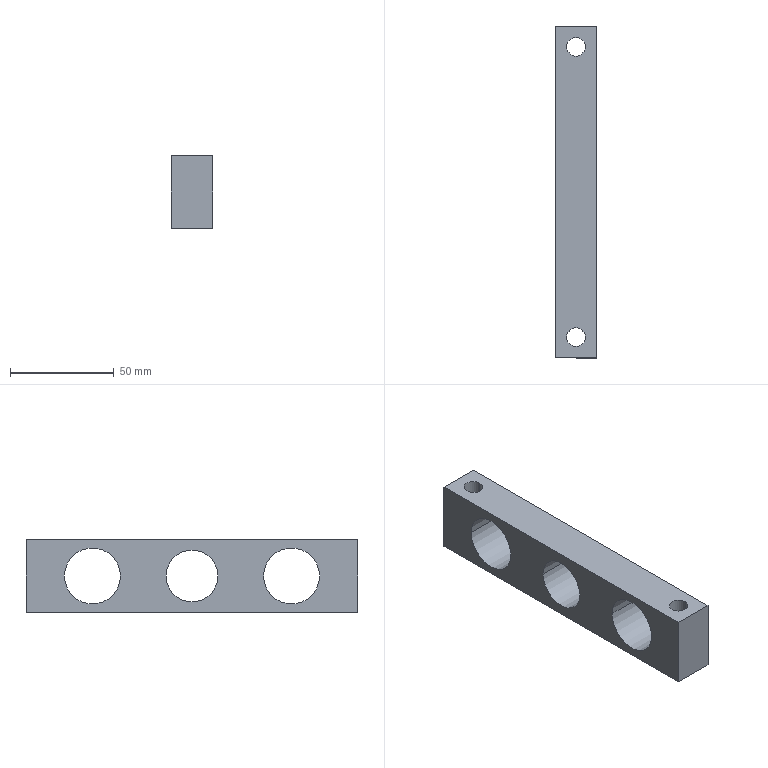Component | SolidWorks | ClampingAssembly-2_CylinderLockingBlock-1 | 1 solid | 22 faces | box 20 x 160 x 35 mm | volume 72882 mm3 | cylinder 14 | plane 8 | commonest cylinder face diameters 15 x4 9 x4 27 x4 25 x2 | material Q235
build123d program:
from build123d import *

# Parameters (mm, degrees)
SKETCH1_W                                       = 160
SKETCH1_H                                       = 35
BOSS_EXTRUDE1_DEPTH                             = 20
SKETCH2_R                                       = 12.5
CUT_EXTRUDE1_DEPTH                              = 85.299
SKETCH3_R                                       = 13.5
CUT_EXTRUDE2_DEPTH                              = 85.299
M8_HEX_SOCKET_HEAD_CAP_SCREW_CBORE1_D           = 9
M8_HEX_SOCKET_HEAD_CAP_SCREW_CBORE1_CBORE_D     = 15
M8_HEX_SOCKET_HEAD_CAP_SCREW_CBORE1_CBORE_DEPTH = 8.6


with BuildPart() as part:
    # Sketch1 → Boss-Extrude1 (new body)
    with BuildSketch(Plane.XY):
        Rectangle(SKETCH1_W, SKETCH1_H)
    extrude(amount=BOSS_EXTRUDE1_DEPTH)

    # Sketch2 → Cut-Extrude1 (cut, through all)
    with BuildSketch(Plane.XY.offset(20)):
        Circle(SKETCH2_R)
    extrude(amount=-CUT_EXTRUDE1_DEPTH, mode=Mode.SUBTRACT)

    # Sketch3 → Cut-Extrude2 (cut, through all)
    with BuildSketch(Plane(origin=(0, 0, 0), x_dir=(-1, 0, 0), z_dir=(0, 0, -1))):
        with Locations((48, 0)):
            Circle(SKETCH3_R)
    cut_extrude2 = extrude(amount=-CUT_EXTRUDE2_DEPTH, mode=Mode.SUBTRACT)

    # Mirror1: Cut-Extrude2 across plane
    add(cut_extrude2.mirror(Plane(origin=(0, 0, 0), x_dir=(0, 0, 1), z_dir=(1, 0, 0))), mode=Mode.SUBTRACT)

    # M8 Hex Socket Head Cap Screw CBORE1 (through all)
    with Locations(Plane(origin=(-70, 17.5, 10), x_dir=(0, 0, 1), z_dir=(0, 1, 0))):
        with Locations((0, 0), (0, 140)):
            CounterBoreHole(M8_HEX_SOCKET_HEAD_CAP_SCREW_CBORE1_D / 2, M8_HEX_SOCKET_HEAD_CAP_SCREW_CBORE1_CBORE_D / 2, M8_HEX_SOCKET_HEAD_CAP_SCREW_CBORE1_CBORE_DEPTH)


solid = part.part

# Placed as in the assembly
solid = solid.moved(Location((-173.215, -26.917, -1210.457), (-90, 90, 0)))
STEP:
#1=COLOUR_RGB('',0.7922,0.8196,0.9333);
#2=FILL_AREA_STYLE_COLOUR('',#1);
#3=FILL_AREA_STYLE('',(#2));
#4=SURFACE_STYLE_FILL_AREA(#3);
#5=SURFACE_SIDE_STYLE('',(#4));
#6=SURFACE_STYLE_USAGE(.BOTH.,#5);
#7=PRESENTATION_STYLE_ASSIGNMENT((#6));
#8=CARTESIAN_POINT('',(-6.721,1.696,-48.006));
#9=VERTEX_POINT('',#8);
#10=CARTESIAN_POINT('',(-6.131,1.696,-48.006));
#11=VERTEX_POINT('',#10);
#12=CARTESIAN_POINT('',(-6.426,1.696,-48.006));
#13=DIRECTION('',(0.,0.,-1.));
#14=DIRECTION('',(1.,-0.,0.));
#15=AXIS2_PLACEMENT_3D('',#12,#13,#14);
#16=CIRCLE('',#15,0.2953);
#17=EDGE_CURVE('',#9,#11,#16,.T.);
#18=ORIENTED_EDGE('',*,*,#17,.F.);
#19=CARTESIAN_POINT('',(-6.721,1.696,-48.345));
#20=VERTEX_POINT('',#19);
#21=CARTESIAN_POINT('',(-6.721,1.696,-48.345));
#22=DIRECTION('',(0.,0.,-1.));
#23=VECTOR('',#22,39.37);
#24=LINE('',#21,#23);
#25=EDGE_CURVE('',#9,#20,#24,.T.);
#26=ORIENTED_EDGE('',*,*,#25,.T.);
#27=CARTESIAN_POINT('',(-6.131,1.696,-48.345));
#28=VERTEX_POINT('',#27);
#29=CARTESIAN_POINT('',(-6.426,1.696,-48.345));
#30=DIRECTION('',(0.,0.,-1.));
#31=DIRECTION('',(1.,-0.,0.));
#32=AXIS2_PLACEMENT_3D('',#29,#30,#31);
#33=CIRCLE('',#32,0.2953);
#34=EDGE_CURVE('',#20,#28,#33,.T.);
#35=ORIENTED_EDGE('',*,*,#34,.T.);
#36=CARTESIAN_POINT('',(-6.131,1.696,-48.345));
#37=DIRECTION('',(0.,0.,-1.));
#38=VECTOR('',#37,39.37);
#39=LINE('',#36,#38);
#40=EDGE_CURVE('',#11,#28,#39,.T.);
#41=ORIENTED_EDGE('',*,*,#40,.F.);
#42=EDGE_LOOP('',(#18,#26,#35,#41));
#43=FACE_OUTER_BOUND('',#42,.T.);
#44=CARTESIAN_POINT('',(-6.426,1.696,-48.345));
#45=DIRECTION('',(0.,0.,-1.));
#46=DIRECTION('',(1.,-0.,0.));
#47=AXIS2_PLACEMENT_3D('',#44,#45,#46);
#48=CYLINDRICAL_SURFACE('',#47,0.2953);
#49=ADVANCED_FACE('',(#43),#48,.F.);
#50=CARTESIAN_POINT('',(-6.603,1.696,-46.967));
#51=VERTEX_POINT('',#50);
#52=CARTESIAN_POINT('',(-6.249,1.696,-46.967));
#53=VERTEX_POINT('',#52);
#54=CARTESIAN_POINT('',(-6.426,1.696,-46.967));
#55=DIRECTION('',(0.,0.,-1.));
#56=DIRECTION('',(1.,0.,0.));
#57=AXIS2_PLACEMENT_3D('',#54,#55,#56);
#58=CIRCLE('',#57,0.1772);
#59=EDGE_CURVE('',#51,#53,#58,.T.);
#60=ORIENTED_EDGE('',*,*,#59,.F.);
#61=CARTESIAN_POINT('',(-6.603,1.696,-48.006));
#62=VERTEX_POINT('',#61);
#63=CARTESIAN_POINT('',(-6.603,1.696,-48.345));
#64=DIRECTION('',(0.,0.,-1.));
#65=VECTOR('',#64,39.37);
#66=LINE('',#63,#65);
#67=EDGE_CURVE('',#51,#62,#66,.T.);
#68=ORIENTED_EDGE('',*,*,#67,.T.);
#69=CARTESIAN_POINT('',(-6.249,1.696,-48.006));
#70=VERTEX_POINT('',#69);
#71=CARTESIAN_POINT('',(-6.426,1.696,-48.006));
#72=DIRECTION('',(0.,0.,-1.));
#73=DIRECTION('',(1.,0.,0.));
#74=AXIS2_PLACEMENT_3D('',#71,#72,#73);
#75=CIRCLE('',#74,0.1772);
#76=EDGE_CURVE('',#62,#70,#75,.T.);
#77=ORIENTED_EDGE('',*,*,#76,.T.);
#78=CARTESIAN_POINT('',(-6.249,1.696,-48.345));
#79=DIRECTION('',(0.,0.,-1.));
#80=VECTOR('',#79,39.37);
#81=LINE('',#78,#80);
#82=EDGE_CURVE('',#53,#70,#81,.T.);
#83=ORIENTED_EDGE('',*,*,#82,.F.);
#84=EDGE_LOOP('',(#60,#68,#77,#83));
#85=FACE_OUTER_BOUND('',#84,.T.);
#86=CARTESIAN_POINT('',(-6.426,1.696,-48.345));
#87=DIRECTION('',(0.,0.,-1.));
#88=DIRECTION('',(1.,0.,0.));
#89=AXIS2_PLACEMENT_3D('',#86,#87,#88);
#90=CYLINDRICAL_SURFACE('',#89,0.1772);
#91=ADVANCED_FACE('',(#85),#90,.F.);
#92=CARTESIAN_POINT('',(-6.721,-3.816,-48.006));
#93=VERTEX_POINT('',#92);
#94=CARTESIAN_POINT('',(-6.131,-3.816,-48.006));
#95=VERTEX_POINT('',#94);
#96=CARTESIAN_POINT('',(-6.426,-3.816,-48.006));
#97=DIRECTION('',(0.,0.,-1.));
#98=DIRECTION('',(1.,0.,0.));
#99=AXIS2_PLACEMENT_3D('',#96,#97,#98);
#100=CIRCLE('',#99,0.2953);
#101=EDGE_CURVE('',#93,#95,#100,.T.);
#102=ORIENTED_EDGE('',*,*,#101,.F.);
#103=CARTESIAN_POINT('',(-6.721,-3.816,-48.345));
#104=VERTEX_POINT('',#103);
#105=CARTESIAN_POINT('',(-6.721,-3.816,-48.345));
#106=DIRECTION('',(0.,0.,-1.));
#107=VECTOR('',#106,39.37);
#108=LINE('',#105,#107);
#109=EDGE_CURVE('',#93,#104,#108,.T.);
#110=ORIENTED_EDGE('',*,*,#109,.T.);
#111=CARTESIAN_POINT('',(-6.131,-3.816,-48.345));
#112=VERTEX_POINT('',#111);
#113=CARTESIAN_POINT('',(-6.426,-3.816,-48.345));
#114=DIRECTION('',(0.,0.,-1.));
#115=DIRECTION('',(1.,0.,0.));
#116=AXIS2_PLACEMENT_3D('',#113,#114,#115);
#117=CIRCLE('',#116,0.2953);
#118=EDGE_CURVE('',#104,#112,#117,.T.);
#119=ORIENTED_EDGE('',*,*,#118,.T.);
#120=CARTESIAN_POINT('',(-6.131,-3.816,-48.345));
#121=DIRECTION('',(0.,0.,-1.));
#122=VECTOR('',#121,39.37);
#123=LINE('',#120,#122);
#124=EDGE_CURVE('',#95,#112,#123,.T.);
#125=ORIENTED_EDGE('',*,*,#124,.F.);
#126=EDGE_LOOP('',(#102,#110,#119,#125));
#127=FACE_OUTER_BOUND('',#126,.T.);
#128=CARTESIAN_POINT('',(-6.426,-3.816,-48.345));
#129=DIRECTION('',(0.,0.,-1.));
#130=DIRECTION('',(1.,0.,0.));
#131=AXIS2_PLACEMENT_3D('',#128,#129,#130);
#132=CYLINDRICAL_SURFACE('',#131,0.2953);
#133=ADVANCED_FACE('',(#127),#132,.F.);
#134=CARTESIAN_POINT('',(-6.603,-3.816,-46.967));
#135=VERTEX_POINT('',#134);
#136=CARTESIAN_POINT('',(-6.249,-3.816,-46.967));
#137=VERTEX_POINT('',#136);
#138=CARTESIAN_POINT('',(-6.426,-3.816,-46.967));
#139=DIRECTION('',(0.,0.,-1.));
#140=DIRECTION('',(1.,0.,0.));
#141=AXIS2_PLACEMENT_3D('',#138,#139,#140);
#142=CIRCLE('',#141,0.1772);
#143=EDGE_CURVE('',#135,#137,#142,.T.);
#144=ORIENTED_EDGE('',*,*,#143,.F.);
#145=CARTESIAN_POINT('',(-6.603,-3.816,-48.006));
#146=VERTEX_POINT('',#145);
#147=CARTESIAN_POINT('',(-6.603,-3.816,-48.345));
#148=DIRECTION('',(0.,0.,-1.));
#149=VECTOR('',#148,39.37);
#150=LINE('',#147,#149);
#151=EDGE_CURVE('',#135,#146,#150,.T.);
#152=ORIENTED_EDGE('',*,*,#151,.T.);
#153=CARTESIAN_POINT('',(-6.249,-3.816,-48.006));
#154=VERTEX_POINT('',#153);
#155=CARTESIAN_POINT('',(-6.426,-3.816,-48.006));
#156=DIRECTION('',(0.,0.,-1.));
#157=DIRECTION('',(1.,0.,0.));
#158=AXIS2_PLACEMENT_3D('',#155,#156,#157);
#159=CIRCLE('',#158,0.1772);
#160=EDGE_CURVE('',#146,#154,#159,.T.);
#161=ORIENTED_EDGE('',*,*,#160,.T.);
#162=CARTESIAN_POINT('',(-6.249,-3.816,-48.345));
#163=DIRECTION('',(0.,0.,-1.));
#164=VECTOR('',#163,39.37);
#165=LINE('',#162,#164);
#166=EDGE_CURVE('',#137,#154,#165,.T.);
#167=ORIENTED_EDGE('',*,*,#166,.F.);
#168=EDGE_LOOP('',(#144,#152,#161,#167));
#169=FACE_OUTER_BOUND('',#168,.T.);
#170=CARTESIAN_POINT('',(-6.426,-3.816,-48.345));
#171=DIRECTION('',(0.,0.,-1.));
#172=DIRECTION('',(1.,0.,0.));
#173=AXIS2_PLACEMENT_3D('',#170,#171,#172);
#174=CYLINDRICAL_SURFACE('',#173,0.1772);
#175=ADVANCED_FACE('',(#169),#174,.F.);
#176=CARTESIAN_POINT('',(-6.032,-2.418,-47.656));
#177=VERTEX_POINT('',#176);
#178=CARTESIAN_POINT('',(-6.032,-3.481,-47.656));
#179=VERTEX_POINT('',#178);
#180=CARTESIAN_POINT('',(-6.032,-2.949,-47.656));
#181=DIRECTION('',(1.,-0.,0.));
#182=DIRECTION('',(0.,-1.,0.));
#183=AXIS2_PLACEMENT_3D('',#180,#181,#182);
#184=CIRCLE('',#183,0.5315);
#185=EDGE_CURVE('',#177,#179,#184,.T.);
#186=ORIENTED_EDGE('',*,*,#185,.T.);
#187=CARTESIAN_POINT('',(-6.819,-3.481,-47.656));
#188=VERTEX_POINT('',#187);
#189=CARTESIAN_POINT('',(-6.032,-3.481,-47.656));
#190=DIRECTION('',(-1.,0.,-0.));
#191=VECTOR('',#190,39.37);
#192=LINE('',#189,#191);
#193=EDGE_CURVE('',#179,#188,#192,.T.);
#194=ORIENTED_EDGE('',*,*,#193,.T.);
#195=CARTESIAN_POINT('',(-6.819,-2.418,-47.656));
#196=VERTEX_POINT('',#195);
#197=CARTESIAN_POINT('',(-6.819,-2.949,-47.656));
#198=DIRECTION('',(1.,-0.,0.));
#199=DIRECTION('',(0.,-1.,0.));
#200=AXIS2_PLACEMENT_3D('',#197,#198,#199);
#201=CIRCLE('',#200,0.5315);
#202=EDGE_CURVE('',#196,#188,#201,.T.);
#203=ORIENTED_EDGE('',*,*,#202,.F.);
#204=CARTESIAN_POINT('',(-6.032,-2.418,-47.656));
#205=DIRECTION('',(-1.,0.,-0.));
#206=VECTOR('',#205,39.37);
#207=LINE('',#204,#206);
#208=EDGE_CURVE('',#177,#196,#207,.T.);
#209=ORIENTED_EDGE('',*,*,#208,.F.);
#210=EDGE_LOOP('',(#186,#194,#203,#209));
#211=FACE_OUTER_BOUND('',#210,.T.);
#212=CARTESIAN_POINT('',(-6.032,-2.949,-47.656));
#213=DIRECTION('',(-1.,0.,-0.));
#214=DIRECTION('',(0.,1.,0.));
#215=AXIS2_PLACEMENT_3D('',#212,#213,#214);
#216=CYLINDRICAL_SURFACE('',#215,0.5315);
#217=ADVANCED_FACE('',(#211),#216,.F.);
#218=CARTESIAN_POINT('',(-6.032,0.2985,-47.656));
#219=VERTEX_POINT('',#218);
#220=CARTESIAN_POINT('',(-6.032,1.362,-47.656));
#221=VERTEX_POINT('',#220);
#222=CARTESIAN_POINT('',(-6.032,0.83,-47.656));
#223=DIRECTION('',(-1.,0.,-0.));
#224=DIRECTION('',(0.,1.,0.));
#225=AXIS2_PLACEMENT_3D('',#222,#223,#224);
#226=CIRCLE('',#225,0.5315);
#227=EDGE_CURVE('',#219,#221,#226,.T.);
#228=ORIENTED_EDGE('',*,*,#227,.F.);
#229=CARTESIAN_POINT('',(-6.819,0.2985,-47.656));
#230=VERTEX_POINT('',#229);
#231=CARTESIAN_POINT('',(-6.032,0.2985,-47.656));
#232=DIRECTION('',(-1.,0.,-0.));
#233=VECTOR('',#232,39.37);
#234=LINE('',#231,#233);
#235=EDGE_CURVE('',#219,#230,#234,.T.);
#236=ORIENTED_EDGE('',*,*,#235,.T.);
#237=CARTESIAN_POINT('',(-6.819,1.362,-47.656));
#238=VERTEX_POINT('',#237);
#239=CARTESIAN_POINT('',(-6.819,0.83,-47.656));
#240=DIRECTION('',(-1.,0.,-0.));
#241=DIRECTION('',(0.,1.,0.));
#242=AXIS2_PLACEMENT_3D('',#239,#240,#241);
#243=CIRCLE('',#242,0.5315);
#244=EDGE_CURVE('',#230,#238,#243,.T.);
#245=ORIENTED_EDGE('',*,*,#244,.T.);
#246=CARTESIAN_POINT('',(-6.032,1.362,-47.656));
#247=DIRECTION('',(-1.,0.,-0.));
#248=VECTOR('',#247,39.37);
#249=LINE('',#246,#248);
#250=EDGE_CURVE('',#221,#238,#249,.T.);
#251=ORIENTED_EDGE('',*,*,#250,.F.);
#252=EDGE_LOOP('',(#228,#236,#245,#251));
#253=FACE_OUTER_BOUND('',#252,.T.);
#254=CARTESIAN_POINT('',(-6.032,0.83,-47.656));
#255=DIRECTION('',(-1.,0.,-0.));
#256=DIRECTION('',(0.,1.,0.));
#257=AXIS2_PLACEMENT_3D('',#254,#255,#256);
#258=CYLINDRICAL_SURFACE('',#257,0.5315);
#259=ADVANCED_FACE('',(#253),#258,.F.);
#260=CARTESIAN_POINT('',(-6.819,-0.5676,-47.656));
#261=VERTEX_POINT('',#260);
#262=CARTESIAN_POINT('',(-6.819,-1.552,-47.656));
#263=VERTEX_POINT('',#262);
#264=CARTESIAN_POINT('',(-6.819,-1.06,-47.656));
#265=DIRECTION('',(1.,-0.,0.));
#266=DIRECTION('',(0.,-1.,0.));
#267=AXIS2_PLACEMENT_3D('',#264,#265,#266);
#268=CIRCLE('',#267,0.4921);
#269=EDGE_CURVE('',#261,#263,#268,.T.);
#270=ORIENTED_EDGE('',*,*,#269,.F.);
#271=CARTESIAN_POINT('',(-6.032,-0.5676,-47.656));
#272=VERTEX_POINT('',#271);
#273=CARTESIAN_POINT('',(-6.819,-0.5676,-47.656));
#274=DIRECTION('',(1.,-0.,0.));
#275=VECTOR('',#274,39.37);
#276=LINE('',#273,#275);
#277=EDGE_CURVE('',#261,#272,#276,.T.);
#278=ORIENTED_EDGE('',*,*,#277,.T.);
#279=CARTESIAN_POINT('',(-6.032,-1.552,-47.656));
#280=VERTEX_POINT('',#279);
#281=CARTESIAN_POINT('',(-6.032,-1.06,-47.656));
#282=DIRECTION('',(1.,-0.,0.));
#283=DIRECTION('',(0.,-1.,0.));
#284=AXIS2_PLACEMENT_3D('',#281,#282,#283);
#285=CIRCLE('',#284,0.4921);
#286=EDGE_CURVE('',#272,#280,#285,.T.);
#287=ORIENTED_EDGE('',*,*,#286,.T.);
#288=CARTESIAN_POINT('',(-6.819,-1.552,-47.656));
#289=DIRECTION('',(1.,-0.,0.));
#290=VECTOR('',#289,39.37);
#291=LINE('',#288,#290);
#292=EDGE_CURVE('',#263,#280,#291,.T.);
#293=ORIENTED_EDGE('',*,*,#292,.F.);
#294=EDGE_LOOP('',(#270,#278,#287,#293));
#295=FACE_OUTER_BOUND('',#294,.T.);
#296=CARTESIAN_POINT('',(-6.819,-1.06,-47.656));
#297=DIRECTION('',(1.,-0.,0.));
#298=DIRECTION('',(0.,-1.,0.));
#299=AXIS2_PLACEMENT_3D('',#296,#297,#298);
#300=CYLINDRICAL_SURFACE('',#299,0.4921);
#301=ADVANCED_FACE('',(#295),#300,.F.);
#302=CARTESIAN_POINT('',(-6.032,-4.209,-46.967));
#303=VERTEX_POINT('',#302);
#304=CARTESIAN_POINT('',(-6.032,-4.209,-48.345));
#305=VERTEX_POINT('',#304);
#306=CARTESIAN_POINT('',(-6.032,-4.209,-48.345));
#307=DIRECTION('',(0.,0.,-1.));
#308=VECTOR('',#307,39.37);
#309=LINE('',#306,#308);
#310=EDGE_CURVE('',#303,#305,#309,.T.);
#311=ORIENTED_EDGE('',*,*,#310,.T.);
#312=CARTESIAN_POINT('',(-6.032,2.09,-48.345));
#313=VERTEX_POINT('',#312);
#314=CARTESIAN_POINT('',(-6.032,2.09,-48.345));
#315=DIRECTION('',(0.,1.,0.));
#316=VECTOR('',#315,39.37);
#317=LINE('',#314,#316);
#318=EDGE_CURVE('',#305,#313,#317,.T.);
#319=ORIENTED_EDGE('',*,*,#318,.T.);
#320=CARTESIAN_POINT('',(-6.032,2.09,-46.967));
#321=VERTEX_POINT('',#320);
#322=CARTESIAN_POINT('',(-6.032,2.09,-48.345));
#323=DIRECTION('',(-0.,-0.,1.));
#324=VECTOR('',#323,39.37);
#325=LINE('',#322,#324);
#326=EDGE_CURVE('',#313,#321,#325,.T.);
#327=ORIENTED_EDGE('',*,*,#326,.T.);
#328=CARTESIAN_POINT('',(-6.032,2.09,-46.967));
#329=DIRECTION('',(-0.,-1.,-0.));
#330=VECTOR('',#329,39.37);
#331=LINE('',#328,#330);
#332=EDGE_CURVE('',#321,#303,#331,.T.);
#333=ORIENTED_EDGE('',*,*,#332,.T.);
#334=EDGE_LOOP('',(#311,#319,#327,#333));
#335=FACE_OUTER_BOUND('',#334,.T.);
#336=CARTESIAN_POINT('',(-6.032,-1.06,-47.656));
#337=DIRECTION('',(1.,-0.,0.));
#338=DIRECTION('',(0.,-1.,0.));
#339=AXIS2_PLACEMENT_3D('',#336,#337,#338);
#340=CIRCLE('',#339,0.4921);
#341=EDGE_CURVE('',#280,#272,#340,.T.);
#342=ORIENTED_EDGE('',*,*,#341,.F.);
#343=ORIENTED_EDGE('',*,*,#286,.F.);
#344=EDGE_LOOP('',(#342,#343));
#345=FACE_BOUND('',#344,.T.);
#346=CARTESIAN_POINT('',(-6.032,0.83,-47.656));
#347=DIRECTION('',(-1.,0.,-0.));
#348=DIRECTION('',(0.,1.,0.));
#349=AXIS2_PLACEMENT_3D('',#346,#347,#348);
#350=CIRCLE('',#349,0.5315);
#351=EDGE_CURVE('',#221,#219,#350,.T.);
#352=ORIENTED_EDGE('',*,*,#351,.T.);
#353=ORIENTED_EDGE('',*,*,#227,.T.);
#354=EDGE_LOOP('',(#352,#353));
#355=FACE_BOUND('',#354,.T.);
#356=ORIENTED_EDGE('',*,*,#185,.F.);
#357=CARTESIAN_POINT('',(-6.032,-2.949,-47.656));
#358=DIRECTION('',(1.,-0.,0.));
#359=DIRECTION('',(0.,-1.,0.));
#360=AXIS2_PLACEMENT_3D('',#357,#358,#359);
#361=CIRCLE('',#360,0.5315);
#362=EDGE_CURVE('',#179,#177,#361,.T.);
#363=ORIENTED_EDGE('',*,*,#362,.F.);
#364=EDGE_LOOP('',(#356,#363));
#365=FACE_BOUND('',#364,.T.);
#366=CARTESIAN_POINT('',(-6.032,-1.06,-47.656));
#367=DIRECTION('',(1.,-0.,0.));
#368=DIRECTION('',(-0.,-1.,-0.));
#369=AXIS2_PLACEMENT_3D('',#366,#367,#368);
#370=PLANE('',#369);
#371=ADVANCED_FACE('',(#335,#345,#355,#365),#370,.T.);
#372=CARTESIAN_POINT('',(-6.819,-4.209,-46.967));
#373=VERTEX_POINT('',#372);
#374=CARTESIAN_POINT('',(-6.819,-4.209,-48.345));
#375=VERTEX_POINT('',#374);
#376=CARTESIAN_POINT('',(-6.819,-4.209,-48.345));
#377=DIRECTION('',(0.,0.,-1.));
#378=VECTOR('',#377,39.37);
#379=LINE('',#376,#378);
#380=EDGE_CURVE('',#373,#375,#379,.T.);
#381=ORIENTED_EDGE('',*,*,#380,.F.);
#382=CARTESIAN_POINT('',(-6.819,2.09,-46.967));
#383=VERTEX_POINT('',#382);
#384=CARTESIAN_POINT('',(-6.819,2.09,-46.967));
#385=DIRECTION('',(-0.,-1.,-0.));
#386=VECTOR('',#385,39.37);
#387=LINE('',#384,#386);
#388=EDGE_CURVE('',#383,#373,#387,.T.);
#389=ORIENTED_EDGE('',*,*,#388,.F.);
#390=CARTESIAN_POINT('',(-6.819,2.09,-48.345));
#391=VERTEX_POINT('',#390);
#392=CARTESIAN_POINT('',(-6.819,2.09,-48.345));
#393=DIRECTION('',(-0.,-0.,1.));
#394=VECTOR('',#393,39.37);
#395=LINE('',#392,#394);
#396=EDGE_CURVE('',#391,#383,#395,.T.);
#397=ORIENTED_EDGE('',*,*,#396,.F.);
#398=CARTESIAN_POINT('',(-6.819,2.09,-48.345));
#399=DIRECTION('',(0.,1.,0.));
#400=VECTOR('',#399,39.37);
#401=LINE('',#398,#400);
#402=EDGE_CURVE('',#375,#391,#401,.T.);
#403=ORIENTED_EDGE('',*,*,#402,.F.);
#404=EDGE_LOOP('',(#381,#389,#397,#403));
#405=FACE_OUTER_BOUND('',#404,.T.);
#406=CARTESIAN_POINT('',(-6.819,-1.06,-47.656));
#407=DIRECTION('',(1.,-0.,0.));
#408=DIRECTION('',(0.,-1.,0.));
#409=AXIS2_PLACEMENT_3D('',#406,#407,#408);
#410=CIRCLE('',#409,0.4921);
#411=EDGE_CURVE('',#263,#261,#410,.T.);
#412=ORIENTED_EDGE('',*,*,#411,.T.);
#413=ORIENTED_EDGE('',*,*,#269,.T.);
#414=EDGE_LOOP('',(#412,#413));
#415=FACE_BOUND('',#414,.T.);
#416=CARTESIAN_POINT('',(-6.819,0.83,-47.656));
#417=DIRECTION('',(-1.,0.,-0.));
#418=DIRECTION('',(0.,1.,0.));
#419=AXIS2_PLACEMENT_3D('',#416,#417,#418);
#420=CIRCLE('',#419,0.5315);
#421=EDGE_CURVE('',#238,#230,#420,.T.);
#422=ORIENTED_EDGE('',*,*,#421,.F.);
#423=ORIENTED_EDGE('',*,*,#244,.F.);
#424=EDGE_LOOP('',(#422,#423));
#425=FACE_BOUND('',#424,.T.);
#426=ORIENTED_EDGE('',*,*,#202,.T.);
#427=CARTESIAN_POINT('',(-6.819,-2.949,-47.656));
#428=DIRECTION('',(1.,-0.,0.));
#429=DIRECTION('',(0.,-1.,0.));
#430=AXIS2_PLACEMENT_3D('',#427,#428,#429);
#431=CIRCLE('',#430,0.5315);
#432=EDGE_CURVE('',#188,#196,#431,.T.);
#433=ORIENTED_EDGE('',*,*,#432,.T.);
#434=EDGE_LOOP('',(#426,#433));
#435=FACE_BOUND('',#434,.T.);
#436=CARTESIAN_POINT('',(-6.819,-1.06,-47.656));
#437=DIRECTION('',(1.,-0.,0.));
#438=DIRECTION('',(-0.,-1.,-0.));
#439=AXIS2_PLACEMENT_3D('',#436,#437,#438);
#440=PLANE('',#439);
#441=ADVANCED_FACE('',(#405,#415,#425,#435),#440,.F.);
#442=ORIENTED_EDGE('',*,*,#380,.T.);
#443=CARTESIAN_POINT('',(-6.032,-4.209,-48.345));
#444=DIRECTION('',(-1.,0.,-0.));
#445=VECTOR('',#444,39.37);
#446=LINE('',#443,#445);
#447=EDGE_CURVE('',#305,#375,#446,.T.);
#448=ORIENTED_EDGE('',*,*,#447,.F.);
#449=ORIENTED_EDGE('',*,*,#310,.F.);
#450=CARTESIAN_POINT('',(-6.032,-4.209,-46.967));
#451=DIRECTION('',(-1.,0.,-0.));
#452=VECTOR('',#451,39.37);
#453=LINE('',#450,#452);
#454=EDGE_CURVE('',#303,#373,#453,.T.);
#455=ORIENTED_EDGE('',*,*,#454,.T.);
#456=EDGE_LOOP('',(#442,#448,#449,#455));
#457=FACE_OUTER_BOUND('',#456,.T.);
#458=CARTESIAN_POINT('',(-6.032,-4.209,-48.345));
#459=DIRECTION('',(0.,1.,0.));
#460=DIRECTION('',(1.,-0.,0.));
#461=AXIS2_PLACEMENT_3D('',#458,#459,#460);
#462=PLANE('',#461);
#463=ADVANCED_FACE('',(#457),#462,.F.);
#464=CARTESIAN_POINT('',(-6.426,1.696,-48.345));
#465=DIRECTION('',(0.,0.,-1.));
#466=DIRECTION('',(1.,-0.,0.));
#467=AXIS2_PLACEMENT_3D('',#464,#465,#466);
#468=CIRCLE('',#467,0.2953);
#469=EDGE_CURVE('',#28,#20,#468,.T.);
#470=ORIENTED_EDGE('',*,*,#469,.F.);
#471=ORIENTED_EDGE('',*,*,#34,.F.);
#472=EDGE_LOOP('',(#470,#471));
#473=FACE_BOUND('',#472,.T.);
#474=CARTESIAN_POINT('',(-6.426,-3.816,-48.345));
#475=DIRECTION('',(0.,0.,-1.));
#476=DIRECTION('',(1.,0.,0.));
#477=AXIS2_PLACEMENT_3D('',#474,#475,#476);
#478=CIRCLE('',#477,0.2953);
#479=EDGE_CURVE('',#112,#104,#478,.T.);
#480=ORIENTED_EDGE('',*,*,#479,.F.);
#481=ORIENTED_EDGE('',*,*,#118,.F.);
#482=EDGE_LOOP('',(#480,#481));
#483=FACE_BOUND('',#482,.T.);
#484=ORIENTED_EDGE('',*,*,#402,.T.);
#485=CARTESIAN_POINT('',(-6.032,2.09,-48.345));
#486=DIRECTION('',(-1.,0.,-0.));
#487=VECTOR('',#486,39.37);
#488=LINE('',#485,#487);
#489=EDGE_CURVE('',#313,#391,#488,.T.);
#490=ORIENTED_EDGE('',*,*,#489,.F.);
#491=ORIENTED_EDGE('',*,*,#318,.F.);
#492=ORIENTED_EDGE('',*,*,#447,.T.);
#493=EDGE_LOOP('',(#484,#490,#491,#492));
#494=FACE_OUTER_BOUND('',#493,.T.);
#495=CARTESIAN_POINT('',(-6.032,2.09,-48.345));
#496=DIRECTION('',(-0.,-0.,1.));
#497=DIRECTION('',(-1.,0.,-0.));
#498=AXIS2_PLACEMENT_3D('',#495,#496,#497);
#499=PLANE('',#498);
#500=ADVANCED_FACE('',(#473,#483,#494),#499,.F.);
#501=ORIENTED_EDGE('',*,*,#396,.T.);
#502=CARTESIAN_POINT('',(-6.032,2.09,-46.967));
#503=DIRECTION('',(-1.,0.,-0.));
#504=VECTOR('',#503,39.37);
#505=LINE('',#502,#504);
#506=EDGE_CURVE('',#321,#383,#505,.T.);
#507=ORIENTED_EDGE('',*,*,#506,.F.);
#508=ORIENTED_EDGE('',*,*,#326,.F.);
#509=ORIENTED_EDGE('',*,*,#489,.T.);
#510=EDGE_LOOP('',(#501,#507,#508,#509));
#511=FACE_OUTER_BOUND('',#510,.T.);
#512=CARTESIAN_POINT('',(-6.032,2.09,-48.345));
#513=DIRECTION('',(-0.,-1.,-0.));
#514=DIRECTION('',(-1.,0.,-0.));
#515=AXIS2_PLACEMENT_3D('',#512,#513,#514);
#516=PLANE('',#515);
#517=ADVANCED_FACE('',(#511),#516,.F.);
#518=CARTESIAN_POINT('',(-6.426,1.696,-46.967));
#519=DIRECTION('',(0.,0.,-1.));
#520=DIRECTION('',(1.,0.,0.));
#521=AXIS2_PLACEMENT_3D('',#518,#519,#520);
#522=CIRCLE('',#521,0.1772);
#523=EDGE_CURVE('',#53,#51,#522,.T.);
#524=ORIENTED_EDGE('',*,*,#523,.T.);
#525=ORIENTED_EDGE('',*,*,#59,.T.);
#526=EDGE_LOOP('',(#524,#525));
#527=FACE_BOUND('',#526,.T.);
#528=CARTESIAN_POINT('',(-6.426,-3.816,-46.967));
#529=DIRECTION('',(0.,0.,-1.));
#530=DIRECTION('',(1.,0.,0.));
#531=AXIS2_PLACEMENT_3D('',#528,#529,#530);
#532=CIRCLE('',#531,0.1772);
#533=EDGE_CURVE('',#137,#135,#532,.T.);
#534=ORIENTED_EDGE('',*,*,#533,.T.);
#535=ORIENTED_EDGE('',*,*,#143,.T.);
#536=EDGE_LOOP('',(#534,#535));
#537=FACE_BOUND('',#536,.T.);
#538=ORIENTED_EDGE('',*,*,#388,.T.);
#539=ORIENTED_EDGE('',*,*,#454,.F.);
#540=ORIENTED_EDGE('',*,*,#332,.F.);
#541=ORIENTED_EDGE('',*,*,#506,.T.);
#542=EDGE_LOOP('',(#538,#539,#540,#541));
#543=FACE_OUTER_BOUND('',#542,.T.);
#544=CARTESIAN_POINT('',(-6.032,2.09,-46.967));
#545=DIRECTION('',(0.,0.,-1.));
#546=DIRECTION('',(1.,-0.,0.));
#547=AXIS2_PLACEMENT_3D('',#544,#545,#546);
#548=PLANE('',#547);
#549=ADVANCED_FACE('',(#527,#537,#543),#548,.F.);
#550=ORIENTED_EDGE('',*,*,#277,.F.);
#551=ORIENTED_EDGE('',*,*,#411,.F.);
#552=ORIENTED_EDGE('',*,*,#292,.T.);
#553=ORIENTED_EDGE('',*,*,#341,.T.);
#554=EDGE_LOOP('',(#550,#551,#552,#553));
#555=FACE_OUTER_BOUND('',#554,.T.);
#556=CARTESIAN_POINT('',(-6.819,-1.06,-47.656));
#557=DIRECTION('',(1.,-0.,0.));
#558=DIRECTION('',(0.,-1.,0.));
#559=AXIS2_PLACEMENT_3D('',#556,#557,#558);
#560=CYLINDRICAL_SURFACE('',#559,0.4921);
#561=ADVANCED_FACE('',(#555),#560,.F.);
#562=ORIENTED_EDGE('',*,*,#235,.F.);
#563=ORIENTED_EDGE('',*,*,#351,.F.);
#564=ORIENTED_EDGE('',*,*,#250,.T.);
#565=ORIENTED_EDGE('',*,*,#421,.T.);
#566=EDGE_LOOP('',(#562,#563,#564,#565));
#567=FACE_OUTER_BOUND('',#566,.T.);
#568=CARTESIAN_POINT('',(-6.032,0.83,-47.656));
#569=DIRECTION('',(-1.,0.,-0.));
#570=DIRECTION('',(0.,1.,0.));
#571=AXIS2_PLACEMENT_3D('',#568,#569,#570);
#572=CYLINDRICAL_SURFACE('',#571,0.5315);
#573=ADVANCED_FACE('',(#567),#572,.F.);
#574=ORIENTED_EDGE('',*,*,#193,.F.);
#575=ORIENTED_EDGE('',*,*,#362,.T.);
#576=ORIENTED_EDGE('',*,*,#208,.T.);
#577=ORIENTED_EDGE('',*,*,#432,.F.);
#578=EDGE_LOOP('',(#574,#575,#576,#577));
#579=FACE_OUTER_BOUND('',#578,.T.);
#580=CARTESIAN_POINT('',(-6.032,-2.949,-47.656));
#581=DIRECTION('',(-1.,0.,-0.));
#582=DIRECTION('',(0.,1.,0.));
#583=AXIS2_PLACEMENT_3D('',#580,#581,#582);
#584=CYLINDRICAL_SURFACE('',#583,0.5315);
#585=ADVANCED_FACE('',(#579),#584,.F.);
#586=ORIENTED_EDGE('',*,*,#151,.F.);
#587=ORIENTED_EDGE('',*,*,#533,.F.);
#588=ORIENTED_EDGE('',*,*,#166,.T.);
#589=CARTESIAN_POINT('',(-6.426,-3.816,-48.006));
#590=DIRECTION('',(0.,0.,-1.));
#591=DIRECTION('',(1.,0.,0.));
#592=AXIS2_PLACEMENT_3D('',#589,#590,#591);
#593=CIRCLE('',#592,0.1772);
#594=EDGE_CURVE('',#154,#146,#593,.T.);
#595=ORIENTED_EDGE('',*,*,#594,.T.);
#596=EDGE_LOOP('',(#586,#587,#588,#595));
#597=FACE_OUTER_BOUND('',#596,.T.);
#598=CARTESIAN_POINT('',(-6.426,-3.816,-48.345));
#599=DIRECTION('',(0.,0.,-1.));
#600=DIRECTION('',(1.,0.,0.));
#601=AXIS2_PLACEMENT_3D('',#598,#599,#600);
#602=CYLINDRICAL_SURFACE('',#601,0.1772);
#603=ADVANCED_FACE('',(#597),#602,.F.);
#604=ORIENTED_EDGE('',*,*,#594,.F.);
#605=ORIENTED_EDGE('',*,*,#160,.F.);
#606=EDGE_LOOP('',(#604,#605));
#607=FACE_BOUND('',#606,.T.);
#608=CARTESIAN_POINT('',(-6.426,-3.816,-48.006));
#609=DIRECTION('',(0.,0.,-1.));
#610=DIRECTION('',(1.,0.,0.));
#611=AXIS2_PLACEMENT_3D('',#608,#609,#610);
#612=CIRCLE('',#611,0.2953);
#613=EDGE_CURVE('',#95,#93,#612,.T.);
#614=ORIENTED_EDGE('',*,*,#613,.T.);
#615=ORIENTED_EDGE('',*,*,#101,.T.);
#616=EDGE_LOOP('',(#614,#615));
#617=FACE_OUTER_BOUND('',#616,.T.);
#618=CARTESIAN_POINT('',(-6.426,-3.993,-48.006));
#619=DIRECTION('',(-0.,-0.,1.));
#620=DIRECTION('',(-1.,0.,-0.));
#621=AXIS2_PLACEMENT_3D('',#618,#619,#620);
#622=PLANE('',#621);
#623=ADVANCED_FACE('',(#607,#617),#622,.F.);
#624=ORIENTED_EDGE('',*,*,#109,.F.);
#625=ORIENTED_EDGE('',*,*,#613,.F.);
#626=ORIENTED_EDGE('',*,*,#124,.T.);
#627=ORIENTED_EDGE('',*,*,#479,.T.);
#628=EDGE_LOOP('',(#624,#625,#626,#627));
#629=FACE_OUTER_BOUND('',#628,.T.);
#630=CARTESIAN_POINT('',(-6.426,-3.816,-48.345));
#631=DIRECTION('',(0.,0.,-1.));
#632=DIRECTION('',(1.,0.,0.));
#633=AXIS2_PLACEMENT_3D('',#630,#631,#632);
#634=CYLINDRICAL_SURFACE('',#633,0.2953);
#635=ADVANCED_FACE('',(#629),#634,.F.);
#636=ORIENTED_EDGE('',*,*,#67,.F.);
#637=ORIENTED_EDGE('',*,*,#523,.F.);
#638=ORIENTED_EDGE('',*,*,#82,.T.);
#639=CARTESIAN_POINT('',(-6.426,1.696,-48.006));
#640=DIRECTION('',(0.,0.,-1.));
#641=DIRECTION('',(1.,0.,0.));
#642=AXIS2_PLACEMENT_3D('',#639,#640,#641);
#643=CIRCLE('',#642,0.1772);
#644=EDGE_CURVE('',#70,#62,#643,.T.);
#645=ORIENTED_EDGE('',*,*,#644,.T.);
#646=EDGE_LOOP('',(#636,#637,#638,#645));
#647=FACE_OUTER_BOUND('',#646,.T.);
#648=CARTESIAN_POINT('',(-6.426,1.696,-48.345));
#649=DIRECTION('',(0.,0.,-1.));
#650=DIRECTION('',(1.,0.,0.));
#651=AXIS2_PLACEMENT_3D('',#648,#649,#650);
#652=CYLINDRICAL_SURFACE('',#651,0.1772);
#653=ADVANCED_FACE('',(#647),#652,.F.);
#654=ORIENTED_EDGE('',*,*,#644,.F.);
#655=ORIENTED_EDGE('',*,*,#76,.F.);
#656=EDGE_LOOP('',(#654,#655));
#657=FACE_BOUND('',#656,.T.);
#658=CARTESIAN_POINT('',(-6.426,1.696,-48.006));
#659=DIRECTION('',(0.,0.,-1.));
#660=DIRECTION('',(1.,-0.,0.));
#661=AXIS2_PLACEMENT_3D('',#658,#659,#660);
#662=CIRCLE('',#661,0.2953);
#663=EDGE_CURVE('',#11,#9,#662,.T.);
#664=ORIENTED_EDGE('',*,*,#663,.T.);
#665=ORIENTED_EDGE('',*,*,#17,.T.);
#666=EDGE_LOOP('',(#664,#665));
#667=FACE_OUTER_BOUND('',#666,.T.);
#668=CARTESIAN_POINT('',(-6.426,1.519,-48.006));
#669=DIRECTION('',(-0.,-0.,1.));
#670=DIRECTION('',(-1.,0.,-0.));
#671=AXIS2_PLACEMENT_3D('',#668,#669,#670);
#672=PLANE('',#671);
#673=ADVANCED_FACE('',(#657,#667),#672,.F.);
#674=ORIENTED_EDGE('',*,*,#25,.F.);
#675=ORIENTED_EDGE('',*,*,#663,.F.);
#676=ORIENTED_EDGE('',*,*,#40,.T.);
#677=ORIENTED_EDGE('',*,*,#469,.T.);
#678=EDGE_LOOP('',(#674,#675,#676,#677));
#679=FACE_OUTER_BOUND('',#678,.T.);
#680=CARTESIAN_POINT('',(-6.426,1.696,-48.345));
#681=DIRECTION('',(0.,0.,-1.));
#682=DIRECTION('',(1.,-0.,0.));
#683=AXIS2_PLACEMENT_3D('',#680,#681,#682);
#684=CYLINDRICAL_SURFACE('',#683,0.2953);
#685=ADVANCED_FACE('',(#679),#684,.F.);
#686=CLOSED_SHELL('',(#49,#91,#133,#175,#217,#259,#301,#371,#441,#463,#500,#517,#549,#561,#573,#585,#603,#623,#635,#653,#673,#685));
#687=MANIFOLD_SOLID_BREP('',#686);
#688=STYLED_ITEM('',(#7),#687);
#689=PRESENTATION_LAYER_ASSIGNMENT('','',(#688));
#690=CARTESIAN_POINT('',(0.,0.,0.));
#691=DIRECTION('',(0.,0.,1.));
#692=DIRECTION('',(1.,0.,0.));
#693=AXIS2_PLACEMENT_3D('',#690,#691,#692);
#694=(LENGTH_UNIT()NAMED_UNIT(*)SI_UNIT($,.METRE.));
#695=LENGTH_MEASURE_WITH_UNIT(LENGTH_MEASURE(0.0254),#694);
#696=DIMENSIONAL_EXPONENTS(1.,0.,0.,0.,0.,0.,0.);
#697=(CONVERSION_BASED_UNIT('',#695)LENGTH_UNIT()NAMED_UNIT(#696));
#698=UNCERTAINTY_MEASURE_WITH_UNIT(LENGTH_MEASURE(0.00001),#697,'','');
#699=(NAMED_UNIT(*)PLANE_ANGLE_UNIT()SI_UNIT($,.RADIAN.));
#700=(NAMED_UNIT(*)SI_UNIT($,.STERADIAN.)SOLID_ANGLE_UNIT());
#701=(GEOMETRIC_REPRESENTATION_CONTEXT(3)GLOBAL_UNCERTAINTY_ASSIGNED_CONTEXT((#698))GLOBAL_UNIT_ASSIGNED_CONTEXT((#697,#699,#700))REPRESENTATION_CONTEXT('',''));
#702=ADVANCED_BREP_SHAPE_REPRESENTATION('',(#687,#693),#701);
#703=(LENGTH_UNIT()NAMED_UNIT(*)SI_UNIT($,.METRE.));
#704=LENGTH_MEASURE_WITH_UNIT(LENGTH_MEASURE(0.0254),#703);
#705=DIMENSIONAL_EXPONENTS(1.,0.,0.,0.,0.,0.,0.);
#706=(CONVERSION_BASED_UNIT('',#704)LENGTH_UNIT()NAMED_UNIT(#705));
#707=UNCERTAINTY_MEASURE_WITH_UNIT(LENGTH_MEASURE(0.00001),#706,'','');
#708=(NAMED_UNIT(*)PLANE_ANGLE_UNIT()SI_UNIT($,.RADIAN.));
#709=(NAMED_UNIT(*)SI_UNIT($,.STERADIAN.)SOLID_ANGLE_UNIT());
#710=(GEOMETRIC_REPRESENTATION_CONTEXT(3)GLOBAL_UNCERTAINTY_ASSIGNED_CONTEXT((#707))GLOBAL_UNIT_ASSIGNED_CONTEXT((#706,#708,#709))REPRESENTATION_CONTEXT('',''));
#711=MECHANICAL_DESIGN_GEOMETRIC_PRESENTATION_REPRESENTATION('',(#688),#710);